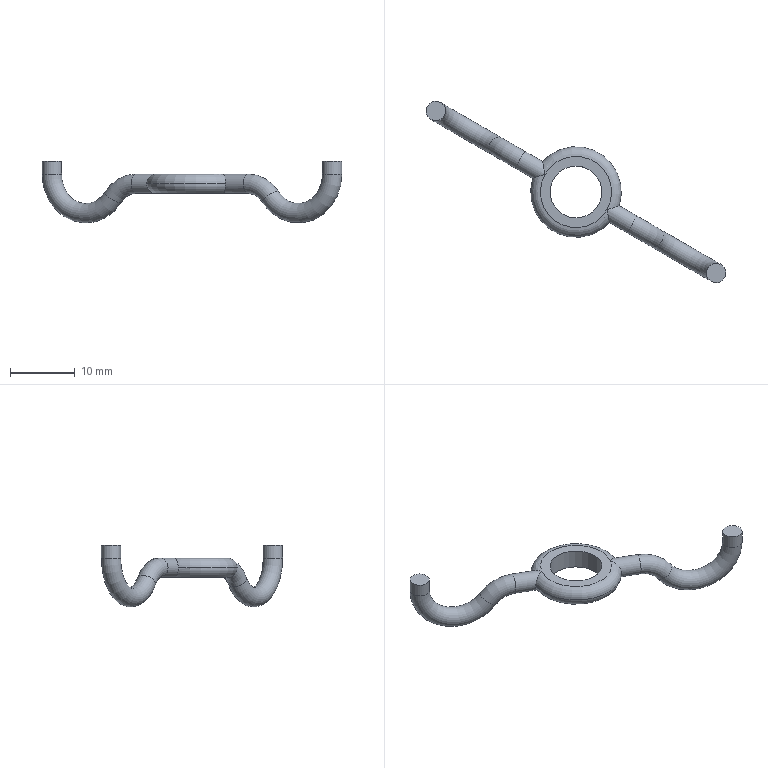Component | NX | LIFTING_RING | 1 solid | 17 faces | volume 627 mm3 | torus 8 | cylinder 5 | plane 4 | commonest cylinder face diameters 3 x4 8 x1